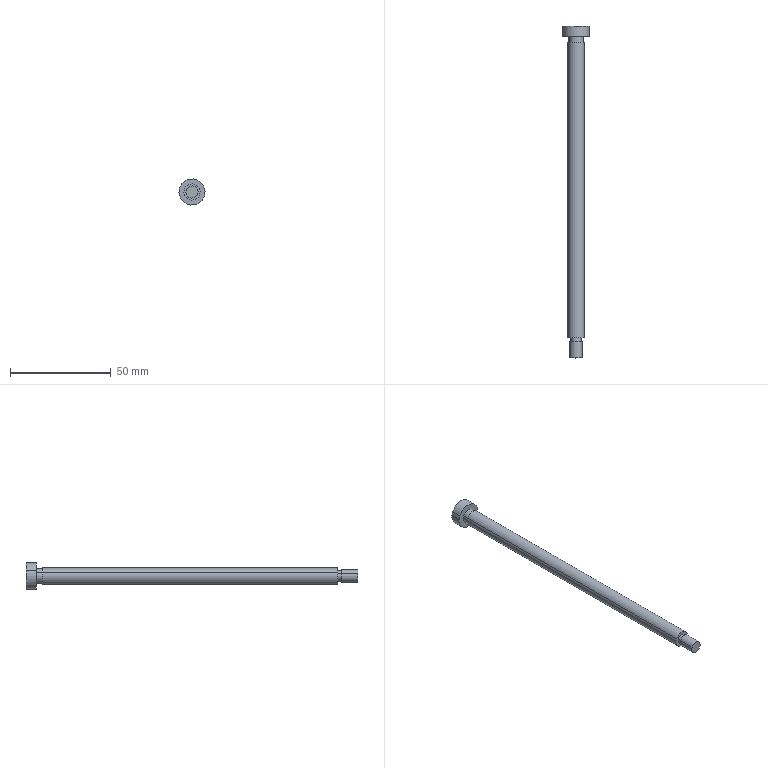Component | SolidWorks | ElectricalBoxAssembly2-1_M6-8-13-150GuidePinBolt-1 | 1 solid | 23 faces | box 13 x 165 x 13 mm | volume 8364 mm3 | plane 13 | cylinder 10 | commonest cylinder face diameters 6 x2 5 x2 13 x2 7 x2 8 x2
STEP:
#1=CARTESIAN_POINT('',(28.077,14.947,60.043));
#2=VERTEX_POINT('',#1);
#3=CARTESIAN_POINT('',(27.865,14.947,60.146));
#4=VERTEX_POINT('',#3);
#5=CARTESIAN_POINT('',(27.971,14.947,60.094));
#6=DIRECTION('',(0.,-1.,-0.));
#7=DIRECTION('',(0.8986,0.,-0.4387));
#8=AXIS2_PLACEMENT_3D('',#5,#6,#7);
#9=CIRCLE('',#8,0.1181);
#10=EDGE_CURVE('',#2,#4,#9,.T.);
#11=ORIENTED_EDGE('',*,*,#10,.F.);
#12=CARTESIAN_POINT('',(28.077,15.262,60.043));
#13=VERTEX_POINT('',#12);
#14=CARTESIAN_POINT('',(28.077,14.947,60.043));
#15=DIRECTION('',(-0.,1.,0.));
#16=VECTOR('',#15,39.37);
#17=LINE('',#14,#16);
#18=EDGE_CURVE('',#2,#13,#17,.T.);
#19=ORIENTED_EDGE('',*,*,#18,.T.);
#20=CARTESIAN_POINT('',(27.865,15.262,60.146));
#21=VERTEX_POINT('',#20);
#22=CARTESIAN_POINT('',(27.971,15.262,60.094));
#23=DIRECTION('',(0.,-1.,-0.));
#24=DIRECTION('',(0.8986,0.,-0.4387));
#25=AXIS2_PLACEMENT_3D('',#22,#23,#24);
#26=CIRCLE('',#25,0.1181);
#27=EDGE_CURVE('',#13,#21,#26,.T.);
#28=ORIENTED_EDGE('',*,*,#27,.T.);
#29=CARTESIAN_POINT('',(27.865,14.947,60.146));
#30=DIRECTION('',(-0.,1.,0.));
#31=VECTOR('',#30,39.37);
#32=LINE('',#29,#31);
#33=EDGE_CURVE('',#4,#21,#32,.T.);
#34=ORIENTED_EDGE('',*,*,#33,.F.);
#35=EDGE_LOOP('',(#11,#19,#28,#34));
#36=FACE_OUTER_BOUND('',#35,.T.);
#37=CARTESIAN_POINT('',(27.971,14.947,60.094));
#38=DIRECTION('',(-0.,1.,0.));
#39=DIRECTION('',(-0.8986,0.,0.4387));
#40=AXIS2_PLACEMENT_3D('',#37,#38,#39);
#41=CYLINDRICAL_SURFACE('',#40,0.1181);
#42=ADVANCED_FACE('',(#36),#41,.T.);
#43=CARTESIAN_POINT('',(28.06,15.262,60.051));
#44=VERTEX_POINT('',#43);
#45=CARTESIAN_POINT('',(27.883,15.262,60.138));
#46=VERTEX_POINT('',#45);
#47=CARTESIAN_POINT('',(27.971,15.262,60.094));
#48=DIRECTION('',(0.,-1.,-0.));
#49=DIRECTION('',(0.8986,0.,-0.4387));
#50=AXIS2_PLACEMENT_3D('',#47,#48,#49);
#51=CIRCLE('',#50,0.09843);
#52=EDGE_CURVE('',#44,#46,#51,.T.);
#53=ORIENTED_EDGE('',*,*,#52,.F.);
#54=CARTESIAN_POINT('',(28.06,15.341,60.051));
#55=VERTEX_POINT('',#54);
#56=CARTESIAN_POINT('',(28.06,15.262,60.051));
#57=DIRECTION('',(-0.,1.,0.));
#58=VECTOR('',#57,39.37);
#59=LINE('',#56,#58);
#60=EDGE_CURVE('',#44,#55,#59,.T.);
#61=ORIENTED_EDGE('',*,*,#60,.T.);
#62=CARTESIAN_POINT('',(27.883,15.341,60.138));
#63=VERTEX_POINT('',#62);
#64=CARTESIAN_POINT('',(27.971,15.341,60.094));
#65=DIRECTION('',(0.,-1.,-0.));
#66=DIRECTION('',(0.8986,0.,-0.4387));
#67=AXIS2_PLACEMENT_3D('',#64,#65,#66);
#68=CIRCLE('',#67,0.09843);
#69=EDGE_CURVE('',#55,#63,#68,.T.);
#70=ORIENTED_EDGE('',*,*,#69,.T.);
#71=CARTESIAN_POINT('',(27.883,15.262,60.138));
#72=DIRECTION('',(-0.,1.,0.));
#73=VECTOR('',#72,39.37);
#74=LINE('',#71,#73);
#75=EDGE_CURVE('',#46,#63,#74,.T.);
#76=ORIENTED_EDGE('',*,*,#75,.F.);
#77=EDGE_LOOP('',(#53,#61,#70,#76));
#78=FACE_OUTER_BOUND('',#77,.T.);
#79=CARTESIAN_POINT('',(27.971,15.262,60.094));
#80=DIRECTION('',(-0.,1.,0.));
#81=DIRECTION('',(-0.8986,0.,0.4387));
#82=AXIS2_PLACEMENT_3D('',#79,#80,#81);
#83=CYLINDRICAL_SURFACE('',#82,0.09843);
#84=ADVANCED_FACE('',(#78),#83,.T.);
#85=CARTESIAN_POINT('',(27.741,21.247,60.207));
#86=VERTEX_POINT('',#85);
#87=CARTESIAN_POINT('',(28.201,21.247,59.982));
#88=VERTEX_POINT('',#87);
#89=CARTESIAN_POINT('',(27.971,21.247,60.094));
#90=DIRECTION('',(-0.,1.,0.));
#91=DIRECTION('',(-0.8986,0.,0.4387));
#92=AXIS2_PLACEMENT_3D('',#89,#90,#91);
#93=CIRCLE('',#92,0.2559);
#94=EDGE_CURVE('',#86,#88,#93,.T.);
#95=ORIENTED_EDGE('',*,*,#94,.T.);
#96=CARTESIAN_POINT('',(28.201,21.444,59.982));
#97=VERTEX_POINT('',#96);
#98=CARTESIAN_POINT('',(28.201,21.247,59.982));
#99=DIRECTION('',(-0.,1.,0.));
#100=VECTOR('',#99,39.37);
#101=LINE('',#98,#100);
#102=EDGE_CURVE('',#88,#97,#101,.T.);
#103=ORIENTED_EDGE('',*,*,#102,.T.);
#104=CARTESIAN_POINT('',(27.741,21.444,60.207));
#105=VERTEX_POINT('',#104);
#106=CARTESIAN_POINT('',(27.971,21.444,60.094));
#107=DIRECTION('',(-0.,1.,0.));
#108=DIRECTION('',(-0.8986,0.,0.4387));
#109=AXIS2_PLACEMENT_3D('',#106,#107,#108);
#110=CIRCLE('',#109,0.2559);
#111=EDGE_CURVE('',#105,#97,#110,.T.);
#112=ORIENTED_EDGE('',*,*,#111,.F.);
#113=CARTESIAN_POINT('',(27.741,21.247,60.207));
#114=DIRECTION('',(-0.,1.,0.));
#115=VECTOR('',#114,39.37);
#116=LINE('',#113,#115);
#117=EDGE_CURVE('',#86,#105,#116,.T.);
#118=ORIENTED_EDGE('',*,*,#117,.F.);
#119=EDGE_LOOP('',(#95,#103,#112,#118));
#120=FACE_OUTER_BOUND('',#119,.T.);
#121=CARTESIAN_POINT('',(27.971,21.247,60.094));
#122=DIRECTION('',(-0.,1.,0.));
#123=DIRECTION('',(-0.8986,0.,0.4387));
#124=AXIS2_PLACEMENT_3D('',#121,#122,#123);
#125=CYLINDRICAL_SURFACE('',#124,0.2559);
#126=ADVANCED_FACE('',(#120),#125,.T.);
#127=CARTESIAN_POINT('',(28.095,21.129,60.034));
#128=VERTEX_POINT('',#127);
#129=CARTESIAN_POINT('',(27.847,21.129,60.155));
#130=VERTEX_POINT('',#129);
#131=CARTESIAN_POINT('',(27.971,21.129,60.094));
#132=DIRECTION('',(0.,-1.,-0.));
#133=DIRECTION('',(0.8986,0.,-0.4387));
#134=AXIS2_PLACEMENT_3D('',#131,#132,#133);
#135=CIRCLE('',#134,0.1378);
#136=EDGE_CURVE('',#128,#130,#135,.T.);
#137=ORIENTED_EDGE('',*,*,#136,.F.);
#138=CARTESIAN_POINT('',(28.095,21.247,60.034));
#139=VERTEX_POINT('',#138);
#140=CARTESIAN_POINT('',(28.095,21.129,60.034));
#141=DIRECTION('',(-0.,1.,0.));
#142=VECTOR('',#141,39.37);
#143=LINE('',#140,#142);
#144=EDGE_CURVE('',#128,#139,#143,.T.);
#145=ORIENTED_EDGE('',*,*,#144,.T.);
#146=CARTESIAN_POINT('',(27.847,21.247,60.155));
#147=VERTEX_POINT('',#146);
#148=CARTESIAN_POINT('',(27.971,21.247,60.094));
#149=DIRECTION('',(0.,-1.,-0.));
#150=DIRECTION('',(0.8986,0.,-0.4387));
#151=AXIS2_PLACEMENT_3D('',#148,#149,#150);
#152=CIRCLE('',#151,0.1378);
#153=EDGE_CURVE('',#139,#147,#152,.T.);
#154=ORIENTED_EDGE('',*,*,#153,.T.);
#155=CARTESIAN_POINT('',(27.847,21.129,60.155));
#156=DIRECTION('',(-0.,1.,0.));
#157=VECTOR('',#156,39.37);
#158=LINE('',#155,#157);
#159=EDGE_CURVE('',#130,#147,#158,.T.);
#160=ORIENTED_EDGE('',*,*,#159,.F.);
#161=EDGE_LOOP('',(#137,#145,#154,#160));
#162=FACE_OUTER_BOUND('',#161,.T.);
#163=CARTESIAN_POINT('',(27.971,21.129,60.094));
#164=DIRECTION('',(-0.,1.,0.));
#165=DIRECTION('',(-0.8986,0.,0.4387));
#166=AXIS2_PLACEMENT_3D('',#163,#164,#165);
#167=CYLINDRICAL_SURFACE('',#166,0.1378);
#168=ADVANCED_FACE('',(#162),#167,.T.);
#169=CARTESIAN_POINT('',(28.113,15.341,60.025));
#170=VERTEX_POINT('',#169);
#171=CARTESIAN_POINT('',(27.83,15.341,60.164));
#172=VERTEX_POINT('',#171);
#173=CARTESIAN_POINT('',(27.971,15.341,60.094));
#174=DIRECTION('',(0.,-1.,-0.));
#175=DIRECTION('',(0.8986,0.,-0.4387));
#176=AXIS2_PLACEMENT_3D('',#173,#174,#175);
#177=CIRCLE('',#176,0.1575);
#178=EDGE_CURVE('',#170,#172,#177,.T.);
#179=ORIENTED_EDGE('',*,*,#178,.F.);
#180=CARTESIAN_POINT('',(28.113,21.129,60.025));
#181=VERTEX_POINT('',#180);
#182=CARTESIAN_POINT('',(28.113,15.341,60.025));
#183=DIRECTION('',(-0.,1.,0.));
#184=VECTOR('',#183,39.37);
#185=LINE('',#182,#184);
#186=EDGE_CURVE('',#170,#181,#185,.T.);
#187=ORIENTED_EDGE('',*,*,#186,.T.);
#188=CARTESIAN_POINT('',(27.83,21.129,60.164));
#189=VERTEX_POINT('',#188);
#190=CARTESIAN_POINT('',(27.971,21.129,60.094));
#191=DIRECTION('',(0.,-1.,-0.));
#192=DIRECTION('',(0.8986,0.,-0.4387));
#193=AXIS2_PLACEMENT_3D('',#190,#191,#192);
#194=CIRCLE('',#193,0.1575);
#195=EDGE_CURVE('',#181,#189,#194,.T.);
#196=ORIENTED_EDGE('',*,*,#195,.T.);
#197=CARTESIAN_POINT('',(27.83,15.341,60.164));
#198=DIRECTION('',(-0.,1.,0.));
#199=VECTOR('',#198,39.37);
#200=LINE('',#197,#199);
#201=EDGE_CURVE('',#172,#189,#200,.T.);
#202=ORIENTED_EDGE('',*,*,#201,.F.);
#203=EDGE_LOOP('',(#179,#187,#196,#202));
#204=FACE_OUTER_BOUND('',#203,.T.);
#205=CARTESIAN_POINT('',(27.971,15.341,60.094));
#206=DIRECTION('',(-0.,1.,0.));
#207=DIRECTION('',(-0.8986,0.,0.4387));
#208=AXIS2_PLACEMENT_3D('',#205,#206,#207);
#209=CYLINDRICAL_SURFACE('',#208,0.1575);
#210=ADVANCED_FACE('',(#204),#209,.T.);
#211=CARTESIAN_POINT('',(27.971,15.341,60.094));
#212=DIRECTION('',(0.,-1.,-0.));
#213=DIRECTION('',(0.8986,0.,-0.4387));
#214=AXIS2_PLACEMENT_3D('',#211,#212,#213);
#215=CIRCLE('',#214,0.1575);
#216=EDGE_CURVE('',#172,#170,#215,.T.);
#217=ORIENTED_EDGE('',*,*,#216,.T.);
#218=ORIENTED_EDGE('',*,*,#178,.T.);
#219=EDGE_LOOP('',(#217,#218));
#220=FACE_OUTER_BOUND('',#219,.T.);
#221=CARTESIAN_POINT('',(27.971,15.341,60.094));
#222=DIRECTION('',(0.,-1.,-0.));
#223=DIRECTION('',(0.8986,0.,-0.4387));
#224=AXIS2_PLACEMENT_3D('',#221,#222,#223);
#225=CIRCLE('',#224,0.09843);
#226=EDGE_CURVE('',#63,#55,#225,.T.);
#227=ORIENTED_EDGE('',*,*,#226,.F.);
#228=ORIENTED_EDGE('',*,*,#69,.F.);
#229=EDGE_LOOP('',(#227,#228));
#230=FACE_BOUND('',#229,.T.);
#231=CARTESIAN_POINT('',(27.971,15.341,60.094));
#232=DIRECTION('',(0.,-1.,-0.));
#233=DIRECTION('',(0.8986,0.,-0.4387));
#234=AXIS2_PLACEMENT_3D('',#231,#232,#233);
#235=PLANE('',#234);
#236=ADVANCED_FACE('',(#220,#230),#235,.T.);
#237=ORIENTED_EDGE('',*,*,#186,.F.);
#238=ORIENTED_EDGE('',*,*,#216,.F.);
#239=ORIENTED_EDGE('',*,*,#201,.T.);
#240=CARTESIAN_POINT('',(27.971,21.129,60.094));
#241=DIRECTION('',(0.,-1.,-0.));
#242=DIRECTION('',(0.8986,0.,-0.4387));
#243=AXIS2_PLACEMENT_3D('',#240,#241,#242);
#244=CIRCLE('',#243,0.1575);
#245=EDGE_CURVE('',#189,#181,#244,.T.);
#246=ORIENTED_EDGE('',*,*,#245,.T.);
#247=EDGE_LOOP('',(#237,#238,#239,#246));
#248=FACE_OUTER_BOUND('',#247,.T.);
#249=CARTESIAN_POINT('',(27.971,15.341,60.094));
#250=DIRECTION('',(-0.,1.,0.));
#251=DIRECTION('',(-0.8986,0.,0.4387));
#252=AXIS2_PLACEMENT_3D('',#249,#250,#251);
#253=CYLINDRICAL_SURFACE('',#252,0.1575);
#254=ADVANCED_FACE('',(#248),#253,.T.);
#255=ORIENTED_EDGE('',*,*,#245,.F.);
#256=ORIENTED_EDGE('',*,*,#195,.F.);
#257=EDGE_LOOP('',(#255,#256));
#258=FACE_OUTER_BOUND('',#257,.T.);
#259=CARTESIAN_POINT('',(27.971,21.129,60.094));
#260=DIRECTION('',(0.,-1.,-0.));
#261=DIRECTION('',(0.8986,0.,-0.4387));
#262=AXIS2_PLACEMENT_3D('',#259,#260,#261);
#263=CIRCLE('',#262,0.1378);
#264=EDGE_CURVE('',#130,#128,#263,.T.);
#265=ORIENTED_EDGE('',*,*,#264,.T.);
#266=ORIENTED_EDGE('',*,*,#136,.T.);
#267=EDGE_LOOP('',(#265,#266));
#268=FACE_BOUND('',#267,.T.);
#269=CARTESIAN_POINT('',(27.971,21.129,60.094));
#270=DIRECTION('',(0.,-1.,-0.));
#271=DIRECTION('',(0.8986,0.,-0.4387));
#272=AXIS2_PLACEMENT_3D('',#269,#270,#271);
#273=PLANE('',#272);
#274=ADVANCED_FACE('',(#258,#268),#273,.F.);
#275=ORIENTED_EDGE('',*,*,#144,.F.);
#276=ORIENTED_EDGE('',*,*,#264,.F.);
#277=ORIENTED_EDGE('',*,*,#159,.T.);
#278=CARTESIAN_POINT('',(27.971,21.247,60.094));
#279=DIRECTION('',(0.,-1.,-0.));
#280=DIRECTION('',(0.8986,0.,-0.4387));
#281=AXIS2_PLACEMENT_3D('',#278,#279,#280);
#282=CIRCLE('',#281,0.1378);
#283=EDGE_CURVE('',#147,#139,#282,.T.);
#284=ORIENTED_EDGE('',*,*,#283,.T.);
#285=EDGE_LOOP('',(#275,#276,#277,#284));
#286=FACE_OUTER_BOUND('',#285,.T.);
#287=CARTESIAN_POINT('',(27.971,21.129,60.094));
#288=DIRECTION('',(-0.,1.,0.));
#289=DIRECTION('',(-0.8986,0.,0.4387));
#290=AXIS2_PLACEMENT_3D('',#287,#288,#289);
#291=CYLINDRICAL_SURFACE('',#290,0.1378);
#292=ADVANCED_FACE('',(#286),#291,.T.);
#293=CARTESIAN_POINT('',(27.896,21.444,60.044));
#294=VERTEX_POINT('',#293);
#295=CARTESIAN_POINT('',(27.889,21.444,60.134));
#296=VERTEX_POINT('',#295);
#297=CARTESIAN_POINT('',(27.896,21.444,60.044));
#298=DIRECTION('',(-0.06935,-0.,0.9976));
#299=VECTOR('',#298,39.37);
#300=LINE('',#297,#299);
#301=EDGE_CURVE('',#294,#296,#300,.T.);
#302=ORIENTED_EDGE('',*,*,#301,.F.);
#303=CARTESIAN_POINT('',(27.977,21.444,60.004));
#304=VERTEX_POINT('',#303);
#305=CARTESIAN_POINT('',(27.977,21.444,60.004));
#306=DIRECTION('',(-0.8986,-0.,0.4387));
#307=VECTOR('',#306,39.37);
#308=LINE('',#305,#307);
#309=EDGE_CURVE('',#304,#294,#308,.T.);
#310=ORIENTED_EDGE('',*,*,#309,.F.);
#311=CARTESIAN_POINT('',(28.053,21.444,60.055));
#312=VERTEX_POINT('',#311);
#313=CARTESIAN_POINT('',(28.053,21.444,60.055));
#314=DIRECTION('',(-0.8293,-0.,-0.5589));
#315=VECTOR('',#314,39.37);
#316=LINE('',#313,#315);
#317=EDGE_CURVE('',#312,#304,#316,.T.);
#318=ORIENTED_EDGE('',*,*,#317,.F.);
#319=CARTESIAN_POINT('',(28.047,21.444,60.145));
#320=VERTEX_POINT('',#319);
#321=CARTESIAN_POINT('',(28.047,21.444,60.145));
#322=DIRECTION('',(0.06935,0.,-0.9976));
#323=VECTOR('',#322,39.37);
#324=LINE('',#321,#323);
#325=EDGE_CURVE('',#320,#312,#324,.T.);
#326=ORIENTED_EDGE('',*,*,#325,.F.);
#327=CARTESIAN_POINT('',(27.965,21.444,60.185));
#328=VERTEX_POINT('',#327);
#329=CARTESIAN_POINT('',(27.965,21.444,60.185));
#330=DIRECTION('',(0.8986,0.,-0.4387));
#331=VECTOR('',#330,39.37);
#332=LINE('',#329,#331);
#333=EDGE_CURVE('',#328,#320,#332,.T.);
#334=ORIENTED_EDGE('',*,*,#333,.F.);
#335=CARTESIAN_POINT('',(27.889,21.444,60.134));
#336=DIRECTION('',(0.8293,0.,0.5589));
#337=VECTOR('',#336,39.37);
#338=LINE('',#335,#337);
#339=EDGE_CURVE('',#296,#328,#338,.T.);
#340=ORIENTED_EDGE('',*,*,#339,.F.);
#341=EDGE_LOOP('',(#302,#310,#318,#326,#334,#340));
#342=FACE_BOUND('',#341,.T.);
#343=ORIENTED_EDGE('',*,*,#111,.T.);
#344=CARTESIAN_POINT('',(27.971,21.444,60.094));
#345=DIRECTION('',(-0.,1.,0.));
#346=DIRECTION('',(-0.8986,0.,0.4387));
#347=AXIS2_PLACEMENT_3D('',#344,#345,#346);
#348=CIRCLE('',#347,0.2559);
#349=EDGE_CURVE('',#97,#105,#348,.T.);
#350=ORIENTED_EDGE('',*,*,#349,.T.);
#351=EDGE_LOOP('',(#343,#350));
#352=FACE_OUTER_BOUND('',#351,.T.);
#353=CARTESIAN_POINT('',(27.971,21.444,60.094));
#354=DIRECTION('',(-0.,1.,0.));
#355=DIRECTION('',(-0.8986,-0.,0.4387));
#356=AXIS2_PLACEMENT_3D('',#353,#354,#355);
#357=PLANE('',#356);
#358=ADVANCED_FACE('',(#342,#352),#357,.T.);
#359=ORIENTED_EDGE('',*,*,#102,.F.);
#360=CARTESIAN_POINT('',(27.971,21.247,60.094));
#361=DIRECTION('',(-0.,1.,0.));
#362=DIRECTION('',(-0.8986,0.,0.4387));
#363=AXIS2_PLACEMENT_3D('',#360,#361,#362);
#364=CIRCLE('',#363,0.2559);
#365=EDGE_CURVE('',#88,#86,#364,.T.);
#366=ORIENTED_EDGE('',*,*,#365,.T.);
#367=ORIENTED_EDGE('',*,*,#117,.T.);
#368=ORIENTED_EDGE('',*,*,#349,.F.);
#369=EDGE_LOOP('',(#359,#366,#367,#368));
#370=FACE_OUTER_BOUND('',#369,.T.);
#371=CARTESIAN_POINT('',(27.971,21.247,60.094));
#372=DIRECTION('',(-0.,1.,0.));
#373=DIRECTION('',(-0.8986,0.,0.4387));
#374=AXIS2_PLACEMENT_3D('',#371,#372,#373);
#375=CYLINDRICAL_SURFACE('',#374,0.2559);
#376=ADVANCED_FACE('',(#370),#375,.T.);
#377=ORIENTED_EDGE('',*,*,#94,.F.);
#378=ORIENTED_EDGE('',*,*,#365,.F.);
#379=EDGE_LOOP('',(#377,#378));
#380=FACE_OUTER_BOUND('',#379,.T.);
#381=ORIENTED_EDGE('',*,*,#283,.F.);
#382=ORIENTED_EDGE('',*,*,#153,.F.);
#383=EDGE_LOOP('',(#381,#382));
#384=FACE_BOUND('',#383,.T.);
#385=CARTESIAN_POINT('',(27.971,21.247,60.094));
#386=DIRECTION('',(-0.,1.,0.));
#387=DIRECTION('',(-0.8986,-0.,0.4387));
#388=AXIS2_PLACEMENT_3D('',#385,#386,#387);
#389=PLANE('',#388);
#390=ADVANCED_FACE('',(#380,#384),#389,.F.);
#391=CARTESIAN_POINT('',(27.971,15.262,60.094));
#392=DIRECTION('',(0.,-1.,-0.));
#393=DIRECTION('',(0.8986,0.,-0.4387));
#394=AXIS2_PLACEMENT_3D('',#391,#392,#393);
#395=CIRCLE('',#394,0.1181);
#396=EDGE_CURVE('',#21,#13,#395,.T.);
#397=ORIENTED_EDGE('',*,*,#396,.F.);
#398=ORIENTED_EDGE('',*,*,#27,.F.);
#399=EDGE_LOOP('',(#397,#398));
#400=FACE_OUTER_BOUND('',#399,.T.);
#401=CARTESIAN_POINT('',(27.971,15.262,60.094));
#402=DIRECTION('',(0.,-1.,-0.));
#403=DIRECTION('',(0.8986,0.,-0.4387));
#404=AXIS2_PLACEMENT_3D('',#401,#402,#403);
#405=CIRCLE('',#404,0.09843);
#406=EDGE_CURVE('',#46,#44,#405,.T.);
#407=ORIENTED_EDGE('',*,*,#406,.T.);
#408=ORIENTED_EDGE('',*,*,#52,.T.);
#409=EDGE_LOOP('',(#407,#408));
#410=FACE_BOUND('',#409,.T.);
#411=CARTESIAN_POINT('',(27.971,15.262,60.094));
#412=DIRECTION('',(0.,-1.,-0.));
#413=DIRECTION('',(0.8986,0.,-0.4387));
#414=AXIS2_PLACEMENT_3D('',#411,#412,#413);
#415=PLANE('',#414);
#416=ADVANCED_FACE('',(#400,#410),#415,.F.);
#417=ORIENTED_EDGE('',*,*,#60,.F.);
#418=ORIENTED_EDGE('',*,*,#406,.F.);
#419=ORIENTED_EDGE('',*,*,#75,.T.);
#420=ORIENTED_EDGE('',*,*,#226,.T.);
#421=EDGE_LOOP('',(#417,#418,#419,#420));
#422=FACE_OUTER_BOUND('',#421,.T.);
#423=CARTESIAN_POINT('',(27.971,15.262,60.094));
#424=DIRECTION('',(-0.,1.,0.));
#425=DIRECTION('',(-0.8986,0.,0.4387));
#426=AXIS2_PLACEMENT_3D('',#423,#424,#425);
#427=CYLINDRICAL_SURFACE('',#426,0.09843);
#428=ADVANCED_FACE('',(#422),#427,.T.);
#429=CARTESIAN_POINT('',(27.971,14.947,60.094));
#430=DIRECTION('',(0.,-1.,-0.));
#431=DIRECTION('',(0.8986,0.,-0.4387));
#432=AXIS2_PLACEMENT_3D('',#429,#430,#431);
#433=CIRCLE('',#432,0.1181);
#434=EDGE_CURVE('',#4,#2,#433,.T.);
#435=ORIENTED_EDGE('',*,*,#434,.T.);
#436=ORIENTED_EDGE('',*,*,#10,.T.);
#437=EDGE_LOOP('',(#435,#436));
#438=FACE_OUTER_BOUND('',#437,.T.);
#439=CARTESIAN_POINT('',(27.971,14.947,60.094));
#440=DIRECTION('',(0.,-1.,-0.));
#441=DIRECTION('',(0.8986,0.,-0.4387));
#442=AXIS2_PLACEMENT_3D('',#439,#440,#441);
#443=PLANE('',#442);
#444=ADVANCED_FACE('',(#438),#443,.T.);
#445=ORIENTED_EDGE('',*,*,#18,.F.);
#446=ORIENTED_EDGE('',*,*,#434,.F.);
#447=ORIENTED_EDGE('',*,*,#33,.T.);
#448=ORIENTED_EDGE('',*,*,#396,.T.);
#449=EDGE_LOOP('',(#445,#446,#447,#448));
#450=FACE_OUTER_BOUND('',#449,.T.);
#451=CARTESIAN_POINT('',(27.971,14.947,60.094));
#452=DIRECTION('',(-0.,1.,0.));
#453=DIRECTION('',(-0.8986,0.,0.4387));
#454=AXIS2_PLACEMENT_3D('',#451,#452,#453);
#455=CYLINDRICAL_SURFACE('',#454,0.1181);
#456=ADVANCED_FACE('',(#450),#455,.T.);
#457=ORIENTED_EDGE('',*,*,#301,.T.);
#458=CARTESIAN_POINT('',(27.889,21.247,60.134));
#459=VERTEX_POINT('',#458);
#460=CARTESIAN_POINT('',(27.889,21.247,60.134));
#461=DIRECTION('',(-0.,1.,0.));
#462=VECTOR('',#461,39.37);
#463=LINE('',#460,#462);
#464=EDGE_CURVE('',#459,#296,#463,.T.);
#465=ORIENTED_EDGE('',*,*,#464,.F.);
#466=CARTESIAN_POINT('',(27.896,21.247,60.044));
#467=VERTEX_POINT('',#466);
#468=CARTESIAN_POINT('',(27.896,21.247,60.044));
#469=DIRECTION('',(-0.06935,-0.,0.9976));
#470=VECTOR('',#469,39.37);
#471=LINE('',#468,#470);
#472=EDGE_CURVE('',#467,#459,#471,.T.);
#473=ORIENTED_EDGE('',*,*,#472,.F.);
#474=CARTESIAN_POINT('',(27.896,21.247,60.044));
#475=DIRECTION('',(-0.,1.,0.));
#476=VECTOR('',#475,39.37);
#477=LINE('',#474,#476);
#478=EDGE_CURVE('',#467,#294,#477,.T.);
#479=ORIENTED_EDGE('',*,*,#478,.T.);
#480=EDGE_LOOP('',(#457,#465,#473,#479));
#481=FACE_OUTER_BOUND('',#480,.T.);
#482=CARTESIAN_POINT('',(27.896,21.247,60.044));
#483=DIRECTION('',(-0.9976,-0.,-0.06935));
#484=DIRECTION('',(-0.06935,-0.,0.9976));
#485=AXIS2_PLACEMENT_3D('',#482,#483,#484);
#486=PLANE('',#485);
#487=ADVANCED_FACE('',(#481),#486,.F.);
#488=ORIENTED_EDGE('',*,*,#309,.T.);
#489=ORIENTED_EDGE('',*,*,#478,.F.);
#490=CARTESIAN_POINT('',(27.977,21.247,60.004));
#491=VERTEX_POINT('',#490);
#492=CARTESIAN_POINT('',(27.977,21.247,60.004));
#493=DIRECTION('',(-0.8986,-0.,0.4387));
#494=VECTOR('',#493,39.37);
#495=LINE('',#492,#494);
#496=EDGE_CURVE('',#491,#467,#495,.T.);
#497=ORIENTED_EDGE('',*,*,#496,.F.);
#498=CARTESIAN_POINT('',(27.977,21.247,60.004));
#499=DIRECTION('',(-0.,1.,0.));
#500=VECTOR('',#499,39.37);
#501=LINE('',#498,#500);
#502=EDGE_CURVE('',#491,#304,#501,.T.);
#503=ORIENTED_EDGE('',*,*,#502,.T.);
#504=EDGE_LOOP('',(#488,#489,#497,#503));
#505=FACE_OUTER_BOUND('',#504,.T.);
#506=CARTESIAN_POINT('',(27.977,21.247,60.004));
#507=DIRECTION('',(-0.4387,0.,-0.8986));
#508=DIRECTION('',(-0.8986,-0.,0.4387));
#509=AXIS2_PLACEMENT_3D('',#506,#507,#508);
#510=PLANE('',#509);
#511=ADVANCED_FACE('',(#505),#510,.F.);
#512=ORIENTED_EDGE('',*,*,#317,.T.);
#513=ORIENTED_EDGE('',*,*,#502,.F.);
#514=CARTESIAN_POINT('',(28.053,21.247,60.055));
#515=VERTEX_POINT('',#514);
#516=CARTESIAN_POINT('',(28.053,21.247,60.055));
#517=DIRECTION('',(-0.8293,-0.,-0.5589));
#518=VECTOR('',#517,39.37);
#519=LINE('',#516,#518);
#520=EDGE_CURVE('',#515,#491,#519,.T.);
#521=ORIENTED_EDGE('',*,*,#520,.F.);
#522=CARTESIAN_POINT('',(28.053,21.247,60.055));
#523=DIRECTION('',(-0.,1.,0.));
#524=VECTOR('',#523,39.37);
#525=LINE('',#522,#524);
#526=EDGE_CURVE('',#515,#312,#525,.T.);
#527=ORIENTED_EDGE('',*,*,#526,.T.);
#528=EDGE_LOOP('',(#512,#513,#521,#527));
#529=FACE_OUTER_BOUND('',#528,.T.);
#530=CARTESIAN_POINT('',(28.053,21.247,60.055));
#531=DIRECTION('',(0.5589,0.,-0.8293));
#532=DIRECTION('',(-0.8293,-0.,-0.5589));
#533=AXIS2_PLACEMENT_3D('',#530,#531,#532);
#534=PLANE('',#533);
#535=ADVANCED_FACE('',(#529),#534,.F.);
#536=ORIENTED_EDGE('',*,*,#325,.T.);
#537=ORIENTED_EDGE('',*,*,#526,.F.);
#538=CARTESIAN_POINT('',(28.047,21.247,60.145));
#539=VERTEX_POINT('',#538);
#540=CARTESIAN_POINT('',(28.047,21.247,60.145));
#541=DIRECTION('',(0.06935,0.,-0.9976));
#542=VECTOR('',#541,39.37);
#543=LINE('',#540,#542);
#544=EDGE_CURVE('',#539,#515,#543,.T.);
#545=ORIENTED_EDGE('',*,*,#544,.F.);
#546=CARTESIAN_POINT('',(28.047,21.247,60.145));
#547=DIRECTION('',(-0.,1.,0.));
#548=VECTOR('',#547,39.37);
#549=LINE('',#546,#548);
#550=EDGE_CURVE('',#539,#320,#549,.T.);
#551=ORIENTED_EDGE('',*,*,#550,.T.);
#552=EDGE_LOOP('',(#536,#537,#545,#551));
#553=FACE_OUTER_BOUND('',#552,.T.);
#554=CARTESIAN_POINT('',(28.047,21.247,60.145));
#555=DIRECTION('',(0.9976,0.,0.06935));
#556=DIRECTION('',(0.06935,0.,-0.9976));
#557=AXIS2_PLACEMENT_3D('',#554,#555,#556);
#558=PLANE('',#557);
#559=ADVANCED_FACE('',(#553),#558,.F.);
#560=ORIENTED_EDGE('',*,*,#333,.T.);
#561=ORIENTED_EDGE('',*,*,#550,.F.);
#562=CARTESIAN_POINT('',(27.965,21.247,60.185));
#563=VERTEX_POINT('',#562);
#564=CARTESIAN_POINT('',(27.965,21.247,60.185));
#565=DIRECTION('',(0.8986,0.,-0.4387));
#566=VECTOR('',#565,39.37);
#567=LINE('',#564,#566);
#568=EDGE_CURVE('',#563,#539,#567,.T.);
#569=ORIENTED_EDGE('',*,*,#568,.F.);
#570=CARTESIAN_POINT('',(27.965,21.247,60.185));
#571=DIRECTION('',(-0.,1.,0.));
#572=VECTOR('',#571,39.37);
#573=LINE('',#570,#572);
#574=EDGE_CURVE('',#563,#328,#573,.T.);
#575=ORIENTED_EDGE('',*,*,#574,.T.);
#576=EDGE_LOOP('',(#560,#561,#569,#575));
#577=FACE_OUTER_BOUND('',#576,.T.);
#578=CARTESIAN_POINT('',(27.965,21.247,60.185));
#579=DIRECTION('',(0.4387,-0.,0.8986));
#580=DIRECTION('',(-0.,1.,0.));
#581=AXIS2_PLACEMENT_3D('',#578,#579,#580);
#582=PLANE('',#581);
#583=ADVANCED_FACE('',(#577),#582,.F.);
#584=ORIENTED_EDGE('',*,*,#339,.T.);
#585=ORIENTED_EDGE('',*,*,#574,.F.);
#586=CARTESIAN_POINT('',(27.889,21.247,60.134));
#587=DIRECTION('',(0.8293,0.,0.5589));
#588=VECTOR('',#587,39.37);
#589=LINE('',#586,#588);
#590=EDGE_CURVE('',#459,#563,#589,.T.);
#591=ORIENTED_EDGE('',*,*,#590,.F.);
#592=ORIENTED_EDGE('',*,*,#464,.T.);
#593=EDGE_LOOP('',(#584,#585,#591,#592));
#594=FACE_OUTER_BOUND('',#593,.T.);
#595=CARTESIAN_POINT('',(27.889,21.247,60.134));
#596=DIRECTION('',(-0.5589,-0.,0.8293));
#597=DIRECTION('',(0.8293,0.,0.5589));
#598=AXIS2_PLACEMENT_3D('',#595,#596,#597);
#599=PLANE('',#598);
#600=ADVANCED_FACE('',(#594),#599,.F.);
#601=ORIENTED_EDGE('',*,*,#472,.T.);
#602=ORIENTED_EDGE('',*,*,#590,.T.);
#603=ORIENTED_EDGE('',*,*,#568,.T.);
#604=ORIENTED_EDGE('',*,*,#544,.T.);
#605=ORIENTED_EDGE('',*,*,#520,.T.);
#606=ORIENTED_EDGE('',*,*,#496,.T.);
#607=EDGE_LOOP('',(#601,#602,#603,#604,#605,#606));
#608=FACE_OUTER_BOUND('',#607,.T.);
#609=CARTESIAN_POINT('',(27.971,21.247,60.094));
#610=DIRECTION('',(-0.,1.,0.));
#611=DIRECTION('',(-0.8986,-0.,0.4387));
#612=AXIS2_PLACEMENT_3D('',#609,#610,#611);
#613=PLANE('',#612);
#614=ADVANCED_FACE('',(#608),#613,.T.);
#615=CLOSED_SHELL('',(#42,#84,#126,#168,#210,#236,#254,#274,#292,#358,#376,#390,#416,#428,#444,#456,#487,#511,#535,#559,#583,#600,#614));
#616=MANIFOLD_SOLID_BREP('',#615);
#617=CARTESIAN_POINT('',(0.,0.,0.));
#618=DIRECTION('',(0.,0.,1.));
#619=DIRECTION('',(1.,0.,0.));
#620=AXIS2_PLACEMENT_3D('',#617,#618,#619);
#621=(LENGTH_UNIT()NAMED_UNIT(*)SI_UNIT($,.METRE.));
#622=LENGTH_MEASURE_WITH_UNIT(LENGTH_MEASURE(0.0254),#621);
#623=DIMENSIONAL_EXPONENTS(1.,0.,0.,0.,0.,0.,0.);
#624=(CONVERSION_BASED_UNIT('',#622)LENGTH_UNIT()NAMED_UNIT(#623));
#625=UNCERTAINTY_MEASURE_WITH_UNIT(LENGTH_MEASURE(0.00001),#624,'','');
#626=(NAMED_UNIT(*)PLANE_ANGLE_UNIT()SI_UNIT($,.RADIAN.));
#627=(NAMED_UNIT(*)SI_UNIT($,.STERADIAN.)SOLID_ANGLE_UNIT());
#628=(GEOMETRIC_REPRESENTATION_CONTEXT(3)GLOBAL_UNCERTAINTY_ASSIGNED_CONTEXT((#625))GLOBAL_UNIT_ASSIGNED_CONTEXT((#624,#626,#627))REPRESENTATION_CONTEXT('',''));
#629=ADVANCED_BREP_SHAPE_REPRESENTATION('',(#616,#620),#628);
#630=COLOUR_RGB('',0.7922,0.8196,0.9333);
#631=FILL_AREA_STYLE_COLOUR('',#630);
#632=FILL_AREA_STYLE('',(#631));
#633=SURFACE_STYLE_FILL_AREA(#632);
#634=SURFACE_SIDE_STYLE('',(#633));
#635=SURFACE_STYLE_USAGE(.BOTH.,#634);
#636=PRESENTATION_STYLE_ASSIGNMENT((#635));
#637=STYLED_ITEM('',(#636),#616);
#638=PRESENTATION_LAYER_ASSIGNMENT('','',(#637));
#639=(LENGTH_UNIT()NAMED_UNIT(*)SI_UNIT($,.METRE.));
#640=LENGTH_MEASURE_WITH_UNIT(LENGTH_MEASURE(0.0254),#639);
#641=DIMENSIONAL_EXPONENTS(1.,0.,0.,0.,0.,0.,0.);
#642=(CONVERSION_BASED_UNIT('',#640)LENGTH_UNIT()NAMED_UNIT(#641));
#643=UNCERTAINTY_MEASURE_WITH_UNIT(LENGTH_MEASURE(0.00001),#642,'','');
#644=(NAMED_UNIT(*)PLANE_ANGLE_UNIT()SI_UNIT($,.RADIAN.));
#645=(NAMED_UNIT(*)SI_UNIT($,.STERADIAN.)SOLID_ANGLE_UNIT());
#646=(GEOMETRIC_REPRESENTATION_CONTEXT(3)GLOBAL_UNCERTAINTY_ASSIGNED_CONTEXT((#643))GLOBAL_UNIT_ASSIGNED_CONTEXT((#642,#644,#645))REPRESENTATION_CONTEXT('',''));
#647=MECHANICAL_DESIGN_GEOMETRIC_PRESENTATION_REPRESENTATION('',(#637),#646);